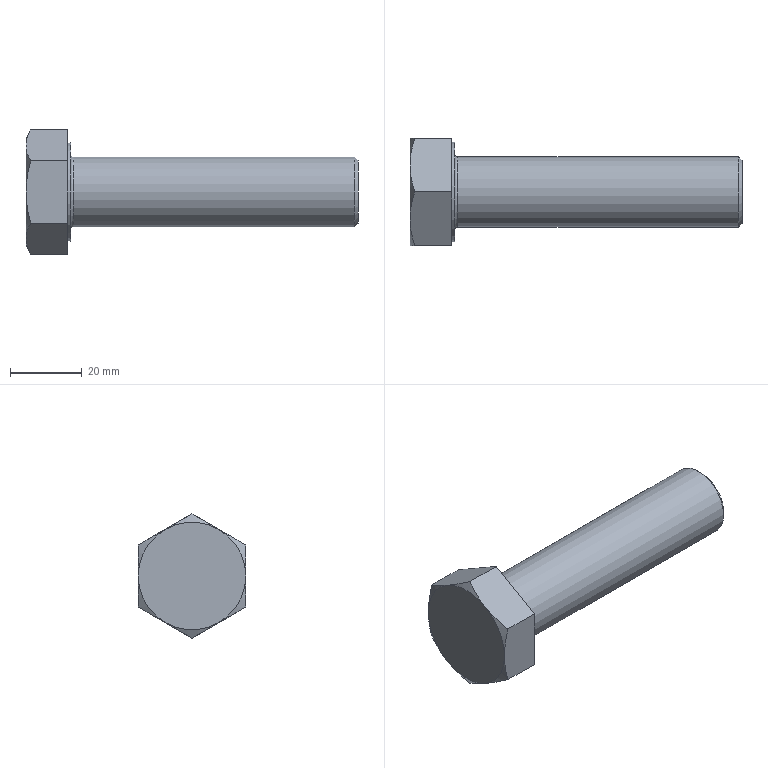Component | NX | GB-T5782-2000_M20X80 | 1 solid | 20 faces | volume 33746 mm3 | plane 10 | cone 7 | cylinder 2 | torus 1 | commonest cylinder face diameters 27.7 x1 19.623 x1